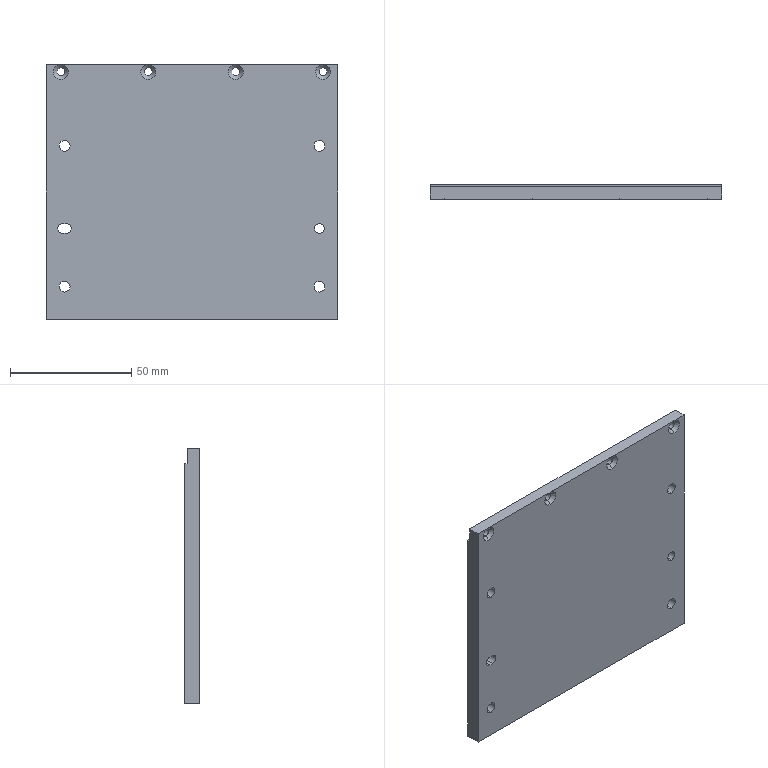CAM job | Mastercam | mm | 17 operations | part box 120 x 6 x 105
1. Contour (Ramp) | 10 - 10 平铣刀
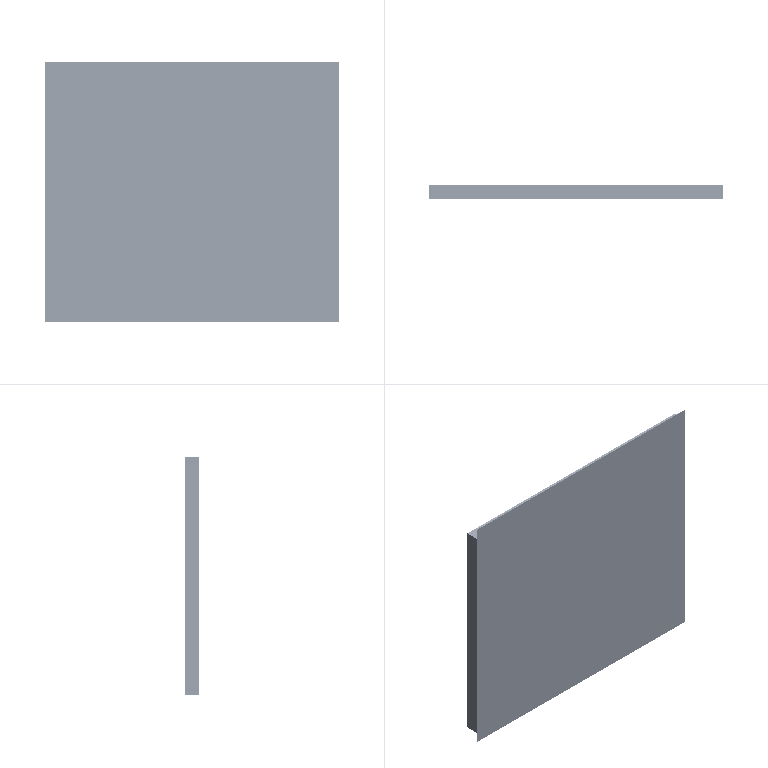2. Contour (2D) | 10 - 10 平铣刀
3. Contour (Ramp) | 10 - 10 平铣刀
4. Contour (2D) | 10 - 10 平铣刀
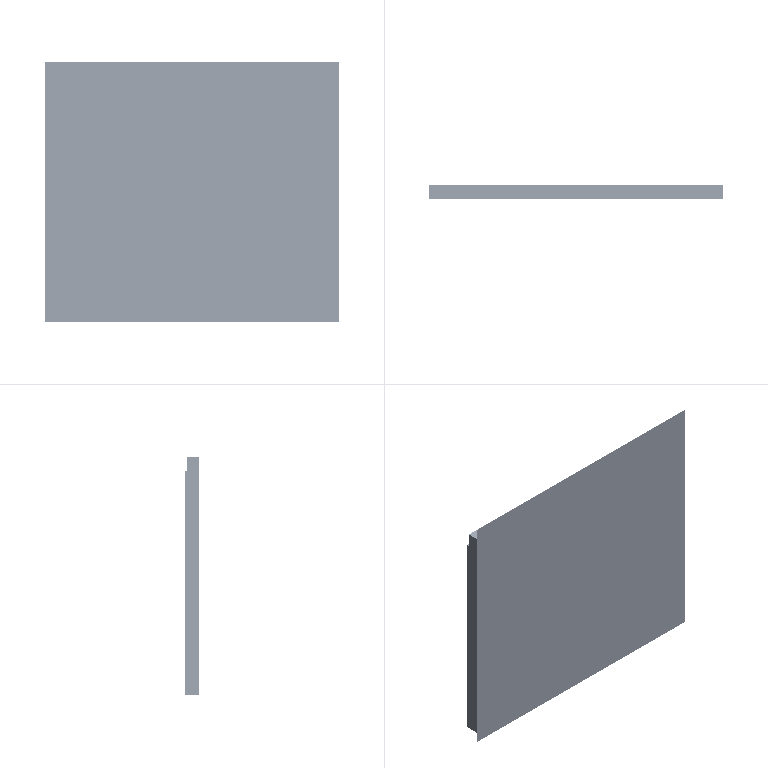5. Contour (Ramp) | 2 - 2 平铣刀
6. Contour (Ramp) | 2 - 2 平铣刀
7. Contour (Ramp) | 4 - 4 平铣刀
8. Contour (2D) | 4 - 4 平铣刀
9. 2D High Speed (2D Area Mill) | 6 - 6 平铣刀
10. Contour (2D) | 6 - 6 平铣刀
11. Contour (2D chamfer) | 7 - 4 倒角刀
12. Contour (2D chamfer) | 7 - 4 倒角刀
13. Drill/Counterbore | 7 - 4 倒角刀
14. Contour (Ramp) | 10 - 10 平铣刀
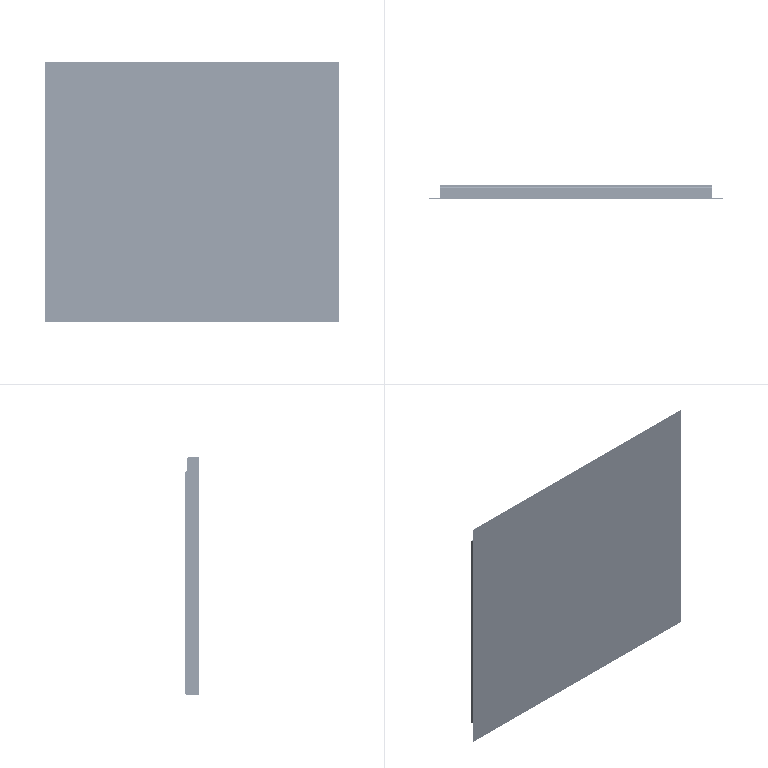15. Contour (2D) | 10 - 10 平铣刀
16. Contour (2D chamfer) | 7 - 4 倒角刀
17. Drill/Counterbore | 7 - 4 倒角刀